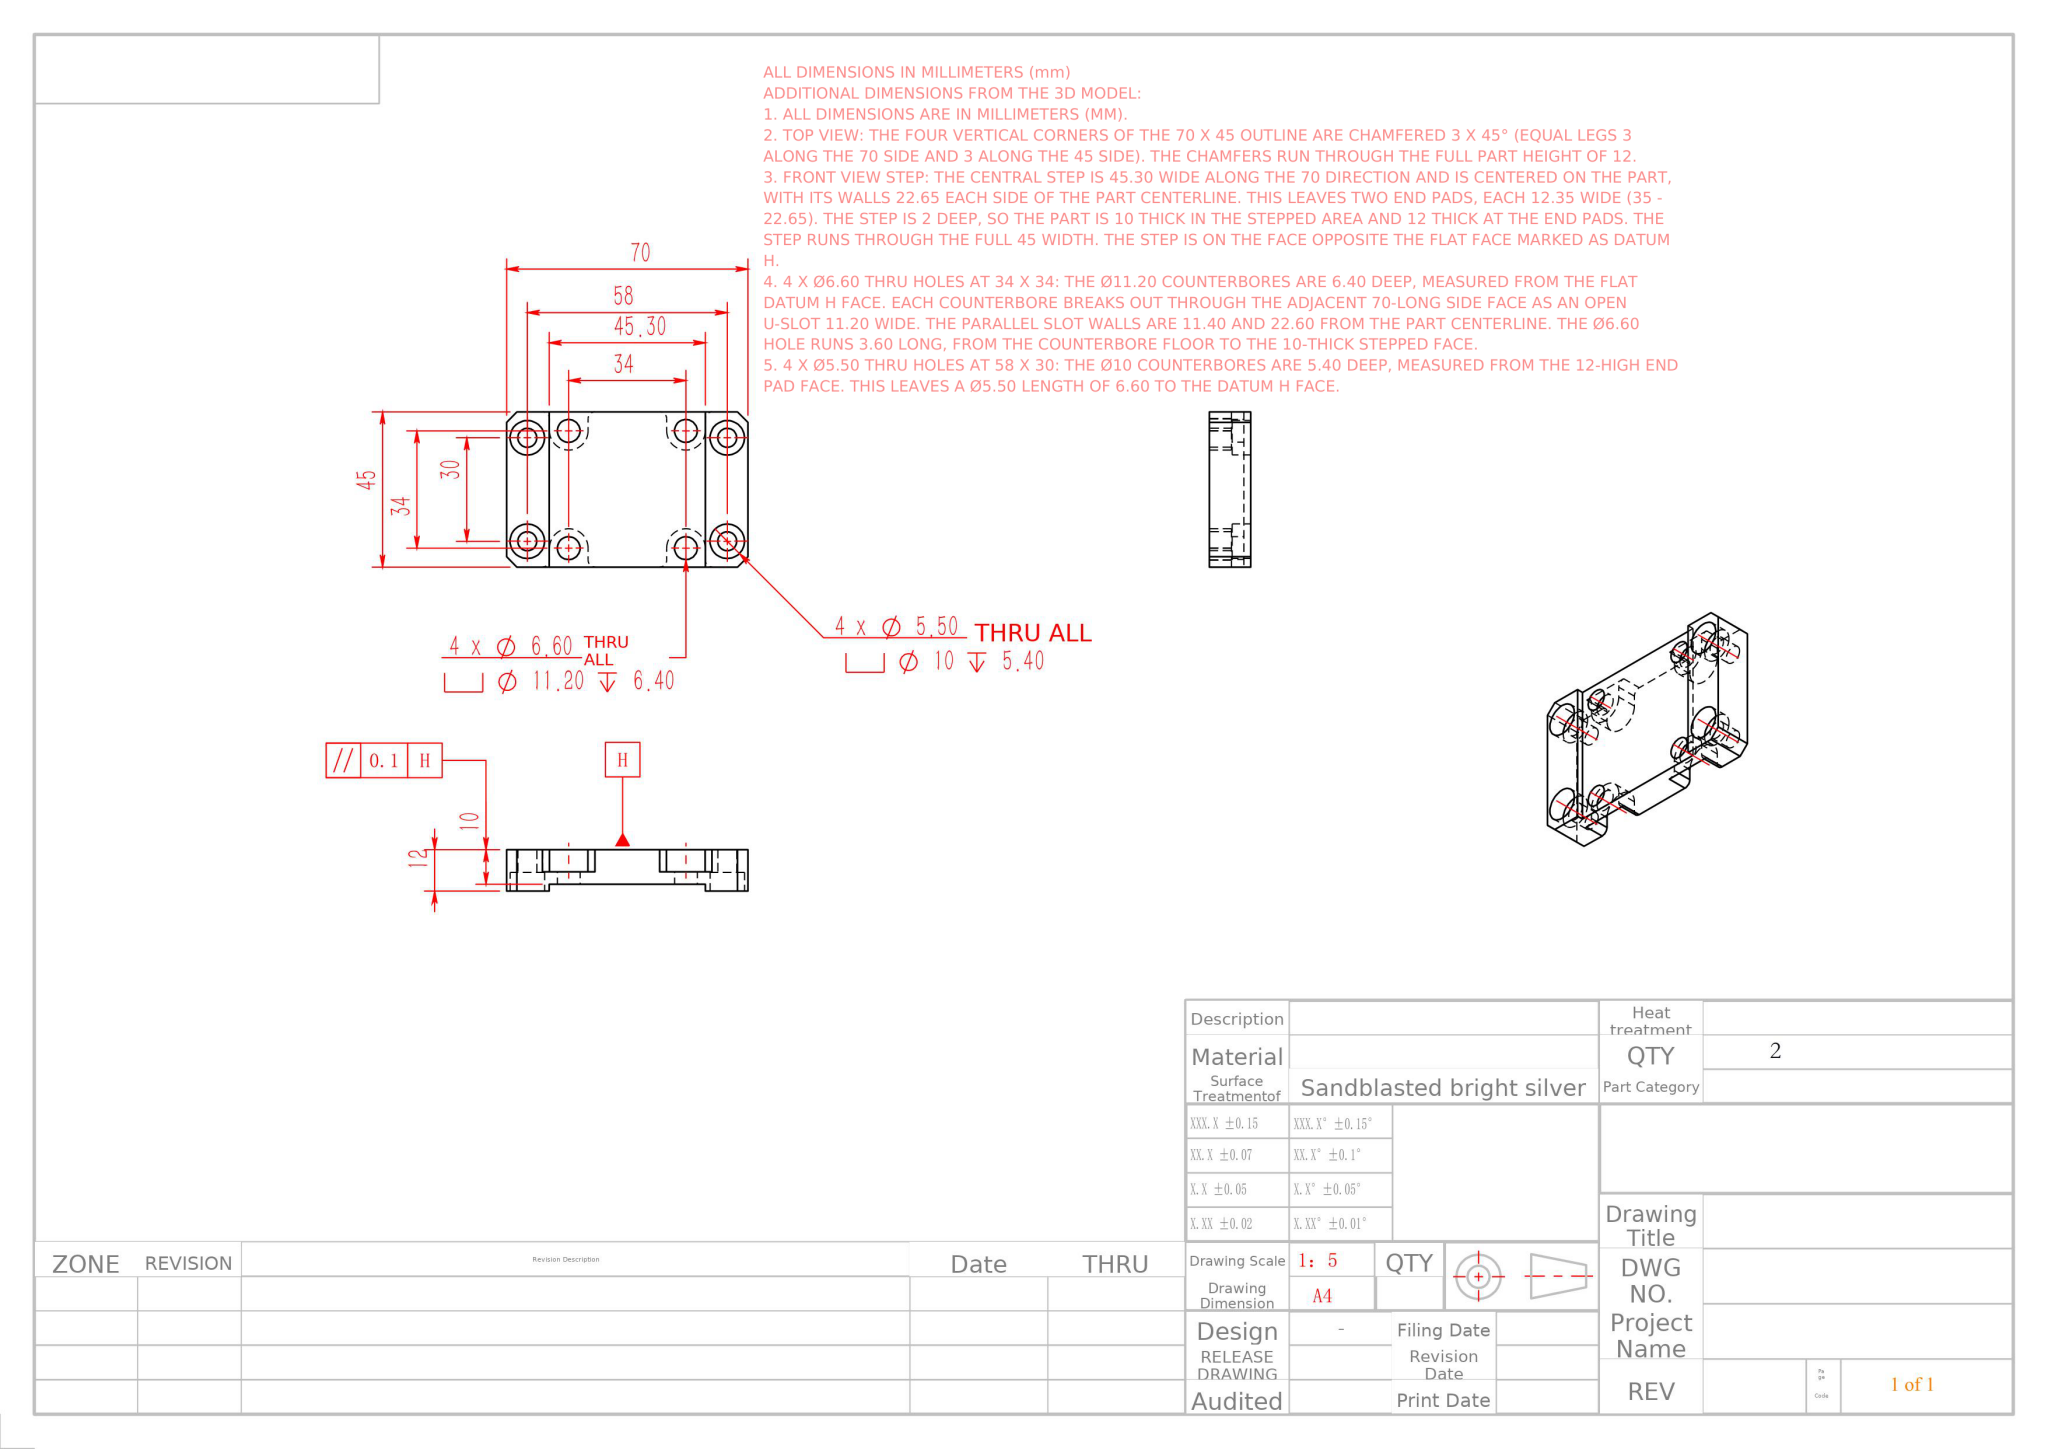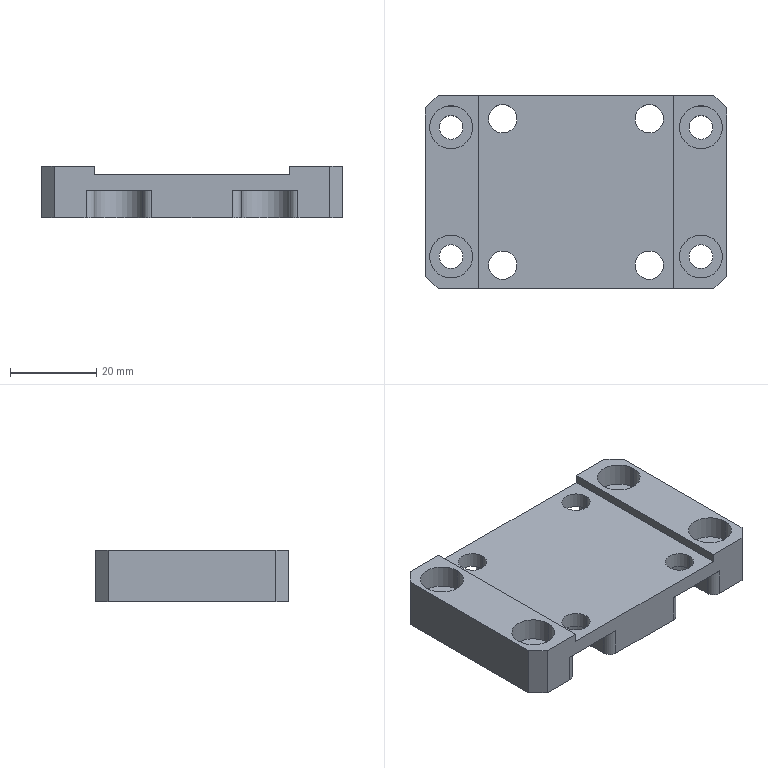Part | NX | mm | Stepped Multi-Bore Adapter Plate 70mm | 1 solid | 66 faces | box 70 x 45 x 12 mm | volume 27809 mm3 | cylinder 36 | plane 30 | commonest cylinder face diameters 6.6 x8 10 x8 5.5 x8 4 x8 11.2 x4